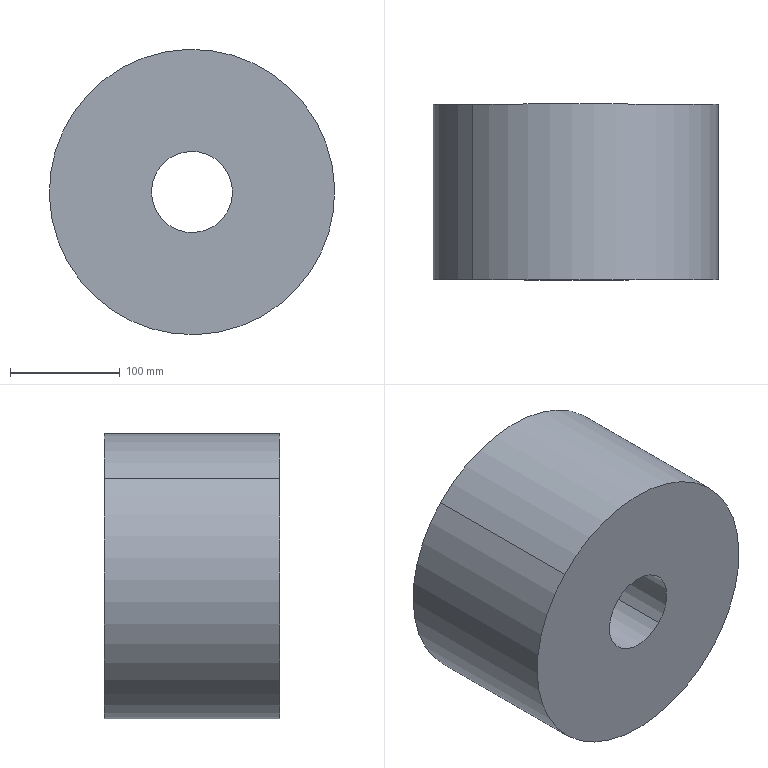Component | SolidWorks | MaterialBarrel-2 | 1 solid | 6 faces | box 260 x 160 x 260 mm | volume 7806732 mm3 | cylinder 4 | plane 2 | commonest cylinder face diameters 74 x2 260 x2
build123d program:
from build123d import *

# Parameters (mm, degrees)
SKETCH1_R           = 130
SKETCH1_R_2         = 37
BOSS_EXTRUDE1_DEPTH = 80


with BuildPart() as part:
    # Sketch1 → Boss-Extrude1 (new, symmetric)
    with BuildSketch(Plane.XY):
        Circle(SKETCH1_R)
        Circle(SKETCH1_R_2, mode=Mode.SUBTRACT)
    extrude(amount=BOSS_EXTRUDE1_DEPTH, both=True)


solid = part.part

# Placed as in the assembly
solid = solid.moved(Location((155, 0, -145), (90, 0, 0)))
STEP:
#1=COLOUR_RGB('',0.7922,0.8196,0.9333);
#2=FILL_AREA_STYLE_COLOUR('',#1);
#3=FILL_AREA_STYLE('',(#2));
#4=SURFACE_STYLE_FILL_AREA(#3);
#5=SURFACE_SIDE_STYLE('',(#4));
#6=SURFACE_STYLE_USAGE(.BOTH.,#5);
#7=PRESENTATION_STYLE_ASSIGNMENT((#6));
#8=CARTESIAN_POINT('',(5.043,3.15,-4.709));
#9=VERTEX_POINT('',#8);
#10=CARTESIAN_POINT('',(7.162,3.15,-6.708));
#11=VERTEX_POINT('',#10);
#12=CARTESIAN_POINT('',(6.102,3.15,-5.709));
#13=DIRECTION('',(-0.,1.,-0.));
#14=DIRECTION('',(0.7273,-0.,-0.6863));
#15=AXIS2_PLACEMENT_3D('',#12,#13,#14);
#16=CIRCLE('',#15,1.457);
#17=EDGE_CURVE('',#9,#11,#16,.T.);
#18=ORIENTED_EDGE('',*,*,#17,.T.);
#19=CARTESIAN_POINT('',(7.162,-3.15,-6.708));
#20=VERTEX_POINT('',#19);
#21=CARTESIAN_POINT('',(7.162,3.15,-6.708));
#22=DIRECTION('',(0.,-1.,0.));
#23=VECTOR('',#22,39.37);
#24=LINE('',#21,#23);
#25=EDGE_CURVE('',#11,#20,#24,.T.);
#26=ORIENTED_EDGE('',*,*,#25,.T.);
#27=CARTESIAN_POINT('',(5.043,-3.15,-4.709));
#28=VERTEX_POINT('',#27);
#29=CARTESIAN_POINT('',(6.102,-3.15,-5.709));
#30=DIRECTION('',(-0.,1.,-0.));
#31=DIRECTION('',(0.7273,-0.,-0.6863));
#32=AXIS2_PLACEMENT_3D('',#29,#30,#31);
#33=CIRCLE('',#32,1.457);
#34=EDGE_CURVE('',#28,#20,#33,.T.);
#35=ORIENTED_EDGE('',*,*,#34,.F.);
#36=CARTESIAN_POINT('',(5.043,3.15,-4.709));
#37=DIRECTION('',(0.,-1.,0.));
#38=VECTOR('',#37,39.37);
#39=LINE('',#36,#38);
#40=EDGE_CURVE('',#9,#28,#39,.T.);
#41=ORIENTED_EDGE('',*,*,#40,.F.);
#42=EDGE_LOOP('',(#18,#26,#35,#41));
#43=FACE_OUTER_BOUND('',#42,.T.);
#44=CARTESIAN_POINT('',(6.102,3.15,-5.709));
#45=DIRECTION('',(0.,-1.,0.));
#46=DIRECTION('',(-0.7273,0.,0.6863));
#47=AXIS2_PLACEMENT_3D('',#44,#45,#46);
#48=CYLINDRICAL_SURFACE('',#47,1.457);
#49=ADVANCED_FACE('',(#43),#48,.F.);
#50=CARTESIAN_POINT('',(9.825,3.15,-9.221));
#51=VERTEX_POINT('',#50);
#52=CARTESIAN_POINT('',(2.38,3.15,-2.196));
#53=VERTEX_POINT('',#52);
#54=CARTESIAN_POINT('',(6.102,3.15,-5.709));
#55=DIRECTION('',(-0.,1.,-0.));
#56=DIRECTION('',(0.7273,-0.,-0.6863));
#57=AXIS2_PLACEMENT_3D('',#54,#55,#56);
#58=CIRCLE('',#57,5.118);
#59=EDGE_CURVE('',#51,#53,#58,.T.);
#60=ORIENTED_EDGE('',*,*,#59,.F.);
#61=CARTESIAN_POINT('',(9.825,-3.15,-9.221));
#62=VERTEX_POINT('',#61);
#63=CARTESIAN_POINT('',(9.825,3.15,-9.221));
#64=DIRECTION('',(0.,-1.,0.));
#65=VECTOR('',#64,39.37);
#66=LINE('',#63,#65);
#67=EDGE_CURVE('',#51,#62,#66,.T.);
#68=ORIENTED_EDGE('',*,*,#67,.T.);
#69=CARTESIAN_POINT('',(2.38,-3.15,-2.196));
#70=VERTEX_POINT('',#69);
#71=CARTESIAN_POINT('',(6.102,-3.15,-5.709));
#72=DIRECTION('',(-0.,1.,-0.));
#73=DIRECTION('',(0.7273,-0.,-0.6863));
#74=AXIS2_PLACEMENT_3D('',#71,#72,#73);
#75=CIRCLE('',#74,5.118);
#76=EDGE_CURVE('',#62,#70,#75,.T.);
#77=ORIENTED_EDGE('',*,*,#76,.T.);
#78=CARTESIAN_POINT('',(2.38,3.15,-2.196));
#79=DIRECTION('',(0.,-1.,0.));
#80=VECTOR('',#79,39.37);
#81=LINE('',#78,#80);
#82=EDGE_CURVE('',#53,#70,#81,.T.);
#83=ORIENTED_EDGE('',*,*,#82,.F.);
#84=EDGE_LOOP('',(#60,#68,#77,#83));
#85=FACE_OUTER_BOUND('',#84,.T.);
#86=CARTESIAN_POINT('',(6.102,3.15,-5.709));
#87=DIRECTION('',(0.,-1.,0.));
#88=DIRECTION('',(-0.7273,0.,0.6863));
#89=AXIS2_PLACEMENT_3D('',#86,#87,#88);
#90=CYLINDRICAL_SURFACE('',#89,5.118);
#91=ADVANCED_FACE('',(#85),#90,.T.);
#92=CARTESIAN_POINT('',(6.102,3.15,-5.709));
#93=DIRECTION('',(-0.,1.,-0.));
#94=DIRECTION('',(0.7273,-0.,-0.6863));
#95=AXIS2_PLACEMENT_3D('',#92,#93,#94);
#96=CIRCLE('',#95,5.118);
#97=EDGE_CURVE('',#53,#51,#96,.T.);
#98=ORIENTED_EDGE('',*,*,#97,.T.);
#99=ORIENTED_EDGE('',*,*,#59,.T.);
#100=EDGE_LOOP('',(#98,#99));
#101=FACE_OUTER_BOUND('',#100,.T.);
#102=ORIENTED_EDGE('',*,*,#17,.F.);
#103=CARTESIAN_POINT('',(6.102,3.15,-5.709));
#104=DIRECTION('',(-0.,1.,-0.));
#105=DIRECTION('',(0.7273,-0.,-0.6863));
#106=AXIS2_PLACEMENT_3D('',#103,#104,#105);
#107=CIRCLE('',#106,1.457);
#108=EDGE_CURVE('',#11,#9,#107,.T.);
#109=ORIENTED_EDGE('',*,*,#108,.F.);
#110=EDGE_LOOP('',(#102,#109));
#111=FACE_BOUND('',#110,.T.);
#112=CARTESIAN_POINT('',(6.102,3.15,-5.709));
#113=DIRECTION('',(-0.,1.,-0.));
#114=DIRECTION('',(0.7273,-0.,-0.6863));
#115=AXIS2_PLACEMENT_3D('',#112,#113,#114);
#116=PLANE('',#115);
#117=ADVANCED_FACE('',(#101,#111),#116,.T.);
#118=CARTESIAN_POINT('',(6.102,-3.15,-5.709));
#119=DIRECTION('',(-0.,1.,-0.));
#120=DIRECTION('',(0.7273,-0.,-0.6863));
#121=AXIS2_PLACEMENT_3D('',#118,#119,#120);
#122=CIRCLE('',#121,5.118);
#123=EDGE_CURVE('',#70,#62,#122,.T.);
#124=ORIENTED_EDGE('',*,*,#123,.F.);
#125=ORIENTED_EDGE('',*,*,#76,.F.);
#126=EDGE_LOOP('',(#124,#125));
#127=FACE_OUTER_BOUND('',#126,.T.);
#128=ORIENTED_EDGE('',*,*,#34,.T.);
#129=CARTESIAN_POINT('',(6.102,-3.15,-5.709));
#130=DIRECTION('',(-0.,1.,-0.));
#131=DIRECTION('',(0.7273,-0.,-0.6863));
#132=AXIS2_PLACEMENT_3D('',#129,#130,#131);
#133=CIRCLE('',#132,1.457);
#134=EDGE_CURVE('',#20,#28,#133,.T.);
#135=ORIENTED_EDGE('',*,*,#134,.T.);
#136=EDGE_LOOP('',(#128,#135));
#137=FACE_BOUND('',#136,.T.);
#138=CARTESIAN_POINT('',(6.102,-3.15,-5.709));
#139=DIRECTION('',(-0.,1.,-0.));
#140=DIRECTION('',(0.7273,-0.,-0.6863));
#141=AXIS2_PLACEMENT_3D('',#138,#139,#140);
#142=PLANE('',#141);
#143=ADVANCED_FACE('',(#127,#137),#142,.F.);
#144=ORIENTED_EDGE('',*,*,#67,.F.);
#145=ORIENTED_EDGE('',*,*,#97,.F.);
#146=ORIENTED_EDGE('',*,*,#82,.T.);
#147=ORIENTED_EDGE('',*,*,#123,.T.);
#148=EDGE_LOOP('',(#144,#145,#146,#147));
#149=FACE_OUTER_BOUND('',#148,.T.);
#150=CARTESIAN_POINT('',(6.102,3.15,-5.709));
#151=DIRECTION('',(0.,-1.,0.));
#152=DIRECTION('',(-0.7273,0.,0.6863));
#153=AXIS2_PLACEMENT_3D('',#150,#151,#152);
#154=CYLINDRICAL_SURFACE('',#153,5.118);
#155=ADVANCED_FACE('',(#149),#154,.T.);
#156=ORIENTED_EDGE('',*,*,#25,.F.);
#157=ORIENTED_EDGE('',*,*,#108,.T.);
#158=ORIENTED_EDGE('',*,*,#40,.T.);
#159=ORIENTED_EDGE('',*,*,#134,.F.);
#160=EDGE_LOOP('',(#156,#157,#158,#159));
#161=FACE_OUTER_BOUND('',#160,.T.);
#162=CARTESIAN_POINT('',(6.102,3.15,-5.709));
#163=DIRECTION('',(0.,-1.,0.));
#164=DIRECTION('',(-0.7273,0.,0.6863));
#165=AXIS2_PLACEMENT_3D('',#162,#163,#164);
#166=CYLINDRICAL_SURFACE('',#165,1.457);
#167=ADVANCED_FACE('',(#161),#166,.F.);
#168=CLOSED_SHELL('',(#49,#91,#117,#143,#155,#167));
#169=MANIFOLD_SOLID_BREP('',#168);
#170=STYLED_ITEM('',(#7),#169);
#171=(LENGTH_UNIT()NAMED_UNIT(*)SI_UNIT($,.METRE.));
#172=LENGTH_MEASURE_WITH_UNIT(LENGTH_MEASURE(0.0254),#171);
#173=DIMENSIONAL_EXPONENTS(1.,0.,0.,0.,0.,0.,0.);
#174=(CONVERSION_BASED_UNIT('',#172)LENGTH_UNIT()NAMED_UNIT(#173));
#175=UNCERTAINTY_MEASURE_WITH_UNIT(LENGTH_MEASURE(0.00001),#174,'','');
#176=(NAMED_UNIT(*)PLANE_ANGLE_UNIT()SI_UNIT($,.RADIAN.));
#177=(NAMED_UNIT(*)SI_UNIT($,.STERADIAN.)SOLID_ANGLE_UNIT());
#178=(GEOMETRIC_REPRESENTATION_CONTEXT(3)GLOBAL_UNCERTAINTY_ASSIGNED_CONTEXT((#175))GLOBAL_UNIT_ASSIGNED_CONTEXT((#174,#176,#177))REPRESENTATION_CONTEXT('',''));
#179=MECHANICAL_DESIGN_GEOMETRIC_PRESENTATION_REPRESENTATION('',(#170),#178);
#180=PRESENTATION_LAYER_ASSIGNMENT('','',(#170));
#181=CARTESIAN_POINT('',(0.,0.,0.));
#182=DIRECTION('',(0.,0.,1.));
#183=DIRECTION('',(1.,0.,0.));
#184=AXIS2_PLACEMENT_3D('',#181,#182,#183);
#185=(LENGTH_UNIT()NAMED_UNIT(*)SI_UNIT($,.METRE.));
#186=LENGTH_MEASURE_WITH_UNIT(LENGTH_MEASURE(0.0254),#185);
#187=DIMENSIONAL_EXPONENTS(1.,0.,0.,0.,0.,0.,0.);
#188=(CONVERSION_BASED_UNIT('',#186)LENGTH_UNIT()NAMED_UNIT(#187));
#189=UNCERTAINTY_MEASURE_WITH_UNIT(LENGTH_MEASURE(0.00001),#188,'','');
#190=(NAMED_UNIT(*)PLANE_ANGLE_UNIT()SI_UNIT($,.RADIAN.));
#191=(NAMED_UNIT(*)SI_UNIT($,.STERADIAN.)SOLID_ANGLE_UNIT());
#192=(GEOMETRIC_REPRESENTATION_CONTEXT(3)GLOBAL_UNCERTAINTY_ASSIGNED_CONTEXT((#189))GLOBAL_UNIT_ASSIGNED_CONTEXT((#188,#190,#191))REPRESENTATION_CONTEXT('',''));
#193=ADVANCED_BREP_SHAPE_REPRESENTATION('',(#169,#184),#192);